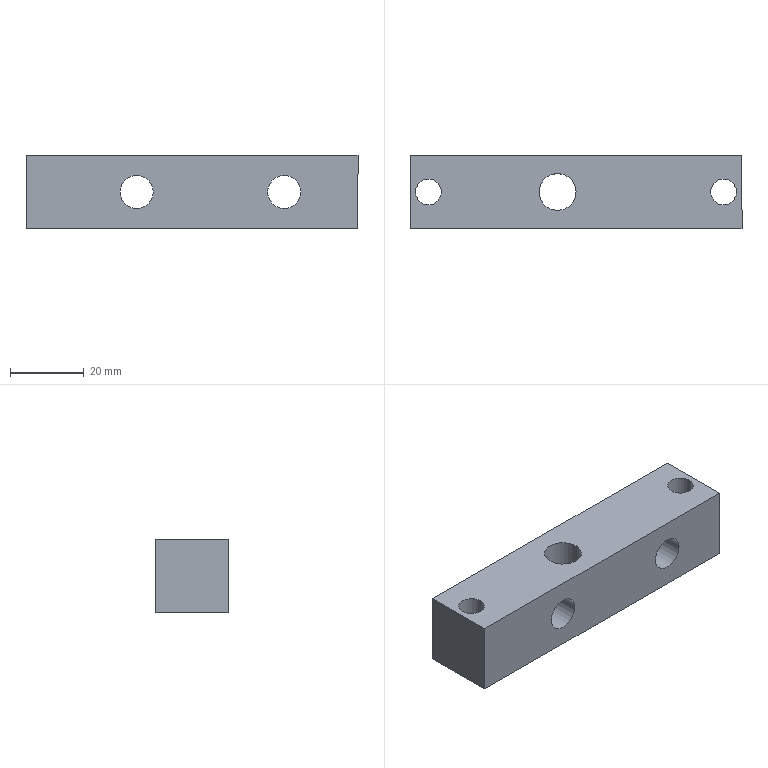Component | SolidWorks | CTM-T-12-AG-02-1 | 1 solid | 16 faces | box 90 x 20 x 20 mm | volume 30345 mm3 | cylinder 10 | plane 6 | commonest cylinder face diameters 7 x4 9 x4 10 x2 | material Q235A
build123d program:
from build123d import *

# Parameters (mm, degrees)
SKETCH1_W                = 20
SKETCH1_H                = 20
BOSS_EXTRUDE1_DEPTH      = 90
M8_CLEARANCE_HOLE1_D     = 9
M8_CLEARANCE_HOLE1_DEPTH = 20
M8_CLEARANCE_HOLE1_TIP   = 2.704
M10_TAPPED_HOLE1_D       = 10
M10_TAPPED_HOLE1_DEPTH   = 27.5
M10_TAPPED_HOLE1_TIP     = 3.004
M6_CLEARANCE_HOLE1_D     = 7
M6_CLEARANCE_HOLE1_DEPTH = 20
M6_CLEARANCE_HOLE1_TIP   = 2.103


with BuildPart() as part:
    # Sketch1 → Boss-Extrude1 (new body)
    with BuildSketch(Plane.XY):
        with Locations((10, 10)):
            Rectangle(SKETCH1_W, SKETCH1_H)
    extrude(amount=BOSS_EXTRUDE1_DEPTH)

    # M8 Clearance Hole1
    with Locations(Plane(origin=(0, 20, 0), x_dir=(-1, 0, 0), z_dir=(0, 1, 0))):
        with Locations((-10, 30), (-10, 70)):
            Hole(M8_CLEARANCE_HOLE1_D / 2, depth=M8_CLEARANCE_HOLE1_DEPTH)
            with Locations((0, 0, -(M8_CLEARANCE_HOLE1_DEPTH + M8_CLEARANCE_HOLE1_TIP / 2))):  # 118° drill point
                Cone(0, M8_CLEARANCE_HOLE1_D / 2, M8_CLEARANCE_HOLE1_TIP, mode=Mode.SUBTRACT)

    # M10 Tapped Hole1
    with Locations(Plane(origin=(20, 0, 0), x_dir=(0, 0, -1), z_dir=(1, 0, 0))):
        with Locations((-40, 10)):
            Hole(M10_TAPPED_HOLE1_D / 2, depth=M10_TAPPED_HOLE1_DEPTH)
            with Locations((0, 0, -(M10_TAPPED_HOLE1_DEPTH + M10_TAPPED_HOLE1_TIP / 2))):  # 118° drill point
                Cone(0, M10_TAPPED_HOLE1_D / 2, M10_TAPPED_HOLE1_TIP, mode=Mode.SUBTRACT)

    # M6 Clearance Hole1
    with Locations(Plane(origin=(20, 0, 0), x_dir=(0, 0, -1), z_dir=(1, 0, 0))):
        with Locations((-85, 10), (-5, 10)):
            Hole(M6_CLEARANCE_HOLE1_D / 2, depth=M6_CLEARANCE_HOLE1_DEPTH)
            with Locations((0, 0, -(M6_CLEARANCE_HOLE1_DEPTH + M6_CLEARANCE_HOLE1_TIP / 2))):  # 118° drill point
                Cone(0, M6_CLEARANCE_HOLE1_D / 2, M6_CLEARANCE_HOLE1_TIP, mode=Mode.SUBTRACT)


solid = part.part

# Placed as in the assembly
solid = solid.moved(Location((0.4, -20, 90), (0, 90, 0)))
STEP:
#1=COLOUR_RGB('',0.7922,0.8196,0.9333);
#2=FILL_AREA_STYLE_COLOUR('',#1);
#3=FILL_AREA_STYLE('',(#2));
#4=SURFACE_STYLE_FILL_AREA(#3);
#5=SURFACE_SIDE_STYLE('',(#4));
#6=SURFACE_STYLE_USAGE(.BOTH.,#5);
#7=PRESENTATION_STYLE_ASSIGNMENT((#6));
#8=CARTESIAN_POINT('',(3.5,-0.3937,2.756));
#9=VERTEX_POINT('',#8);
#10=CARTESIAN_POINT('',(3.224,-0.3937,2.756));
#11=VERTEX_POINT('',#10);
#12=CARTESIAN_POINT('',(3.362,-0.3937,2.756));
#13=DIRECTION('',(0.,-0.,1.));
#14=DIRECTION('',(-1.,0.,0.));
#15=AXIS2_PLACEMENT_3D('',#12,#13,#14);
#16=CIRCLE('',#15,0.1378);
#17=EDGE_CURVE('',#9,#11,#16,.T.);
#18=ORIENTED_EDGE('',*,*,#17,.F.);
#19=CARTESIAN_POINT('',(3.5,-0.3937,3.543));
#20=VERTEX_POINT('',#19);
#21=CARTESIAN_POINT('',(3.5,-0.3937,3.543));
#22=DIRECTION('',(0.,-0.,1.));
#23=VECTOR('',#22,39.37);
#24=LINE('',#21,#23);
#25=EDGE_CURVE('',#9,#20,#24,.T.);
#26=ORIENTED_EDGE('',*,*,#25,.T.);
#27=CARTESIAN_POINT('',(3.224,-0.3937,3.543));
#28=VERTEX_POINT('',#27);
#29=CARTESIAN_POINT('',(3.362,-0.3937,3.543));
#30=DIRECTION('',(0.,-0.,1.));
#31=DIRECTION('',(-1.,0.,0.));
#32=AXIS2_PLACEMENT_3D('',#29,#30,#31);
#33=CIRCLE('',#32,0.1378);
#34=EDGE_CURVE('',#20,#28,#33,.T.);
#35=ORIENTED_EDGE('',*,*,#34,.T.);
#36=CARTESIAN_POINT('',(3.224,-0.3937,3.543));
#37=DIRECTION('',(0.,-0.,1.));
#38=VECTOR('',#37,39.37);
#39=LINE('',#36,#38);
#40=EDGE_CURVE('',#11,#28,#39,.T.);
#41=ORIENTED_EDGE('',*,*,#40,.F.);
#42=EDGE_LOOP('',(#18,#26,#35,#41));
#43=FACE_OUTER_BOUND('',#42,.T.);
#44=CARTESIAN_POINT('',(3.362,-0.3937,3.543));
#45=DIRECTION('',(0.,-0.,1.));
#46=DIRECTION('',(-1.,0.,0.));
#47=AXIS2_PLACEMENT_3D('',#44,#45,#46);
#48=CYLINDRICAL_SURFACE('',#47,0.1378);
#49=ADVANCED_FACE('',(#43),#48,.F.);
#50=CARTESIAN_POINT('',(0.3504,-0.3937,2.756));
#51=VERTEX_POINT('',#50);
#52=CARTESIAN_POINT('',(0.0748,-0.3937,2.756));
#53=VERTEX_POINT('',#52);
#54=CARTESIAN_POINT('',(0.2126,-0.3937,2.756));
#55=DIRECTION('',(0.,-0.,1.));
#56=DIRECTION('',(-1.,0.,0.));
#57=AXIS2_PLACEMENT_3D('',#54,#55,#56);
#58=CIRCLE('',#57,0.1378);
#59=EDGE_CURVE('',#51,#53,#58,.T.);
#60=ORIENTED_EDGE('',*,*,#59,.F.);
#61=CARTESIAN_POINT('',(0.3504,-0.3937,3.543));
#62=VERTEX_POINT('',#61);
#63=CARTESIAN_POINT('',(0.3504,-0.3937,3.543));
#64=DIRECTION('',(0.,-0.,1.));
#65=VECTOR('',#64,39.37);
#66=LINE('',#63,#65);
#67=EDGE_CURVE('',#51,#62,#66,.T.);
#68=ORIENTED_EDGE('',*,*,#67,.T.);
#69=CARTESIAN_POINT('',(0.0748,-0.3937,3.543));
#70=VERTEX_POINT('',#69);
#71=CARTESIAN_POINT('',(0.2126,-0.3937,3.543));
#72=DIRECTION('',(0.,-0.,1.));
#73=DIRECTION('',(-1.,0.,0.));
#74=AXIS2_PLACEMENT_3D('',#71,#72,#73);
#75=CIRCLE('',#74,0.1378);
#76=EDGE_CURVE('',#62,#70,#75,.T.);
#77=ORIENTED_EDGE('',*,*,#76,.T.);
#78=CARTESIAN_POINT('',(0.0748,-0.3937,3.543));
#79=DIRECTION('',(0.,-0.,1.));
#80=VECTOR('',#79,39.37);
#81=LINE('',#78,#80);
#82=EDGE_CURVE('',#53,#70,#81,.T.);
#83=ORIENTED_EDGE('',*,*,#82,.F.);
#84=EDGE_LOOP('',(#60,#68,#77,#83));
#85=FACE_OUTER_BOUND('',#84,.T.);
#86=CARTESIAN_POINT('',(0.2126,-0.3937,3.543));
#87=DIRECTION('',(0.,-0.,1.));
#88=DIRECTION('',(-1.,0.,0.));
#89=AXIS2_PLACEMENT_3D('',#86,#87,#88);
#90=CYLINDRICAL_SURFACE('',#89,0.1378);
#91=ADVANCED_FACE('',(#85),#90,.F.);
#92=CARTESIAN_POINT('',(1.787,-0.3937,2.756));
#93=VERTEX_POINT('',#92);
#94=CARTESIAN_POINT('',(1.394,-0.3937,2.756));
#95=VERTEX_POINT('',#94);
#96=CARTESIAN_POINT('',(1.591,-0.3937,2.756));
#97=DIRECTION('',(0.,-0.,1.));
#98=DIRECTION('',(-1.,-0.,0.));
#99=AXIS2_PLACEMENT_3D('',#96,#97,#98);
#100=CIRCLE('',#99,0.1969);
#101=EDGE_CURVE('',#93,#95,#100,.T.);
#102=ORIENTED_EDGE('',*,*,#101,.F.);
#103=CARTESIAN_POINT('',(1.787,-0.3937,3.543));
#104=VERTEX_POINT('',#103);
#105=CARTESIAN_POINT('',(1.787,-0.3937,3.543));
#106=DIRECTION('',(0.,-0.,1.));
#107=VECTOR('',#106,39.37);
#108=LINE('',#105,#107);
#109=EDGE_CURVE('',#93,#104,#108,.T.);
#110=ORIENTED_EDGE('',*,*,#109,.T.);
#111=CARTESIAN_POINT('',(1.394,-0.3937,3.543));
#112=VERTEX_POINT('',#111);
#113=CARTESIAN_POINT('',(1.591,-0.3937,3.543));
#114=DIRECTION('',(0.,-0.,1.));
#115=DIRECTION('',(-1.,-0.,0.));
#116=AXIS2_PLACEMENT_3D('',#113,#114,#115);
#117=CIRCLE('',#116,0.1969);
#118=EDGE_CURVE('',#104,#112,#117,.T.);
#119=ORIENTED_EDGE('',*,*,#118,.T.);
#120=CARTESIAN_POINT('',(1.394,-0.3937,3.543));
#121=DIRECTION('',(0.,-0.,1.));
#122=VECTOR('',#121,39.37);
#123=LINE('',#120,#122);
#124=EDGE_CURVE('',#95,#112,#123,.T.);
#125=ORIENTED_EDGE('',*,*,#124,.F.);
#126=EDGE_LOOP('',(#102,#110,#119,#125));
#127=FACE_OUTER_BOUND('',#126,.T.);
#128=CARTESIAN_POINT('',(1.591,-0.3937,3.543));
#129=DIRECTION('',(0.,-0.,1.));
#130=DIRECTION('',(-1.,-0.,0.));
#131=AXIS2_PLACEMENT_3D('',#128,#129,#130);
#132=CYLINDRICAL_SURFACE('',#131,0.1969);
#133=ADVANCED_FACE('',(#127),#132,.F.);
#134=CARTESIAN_POINT('',(1.02,0.,3.15));
#135=VERTEX_POINT('',#134);
#136=CARTESIAN_POINT('',(1.374,0.,3.15));
#137=VERTEX_POINT('',#136);
#138=CARTESIAN_POINT('',(1.197,0.,3.15));
#139=DIRECTION('',(0.,-1.,-0.));
#140=DIRECTION('',(1.,0.,0.));
#141=AXIS2_PLACEMENT_3D('',#138,#139,#140);
#142=CIRCLE('',#141,0.1772);
#143=EDGE_CURVE('',#135,#137,#142,.T.);
#144=ORIENTED_EDGE('',*,*,#143,.F.);
#145=CARTESIAN_POINT('',(1.02,-0.7874,3.15));
#146=VERTEX_POINT('',#145);
#147=CARTESIAN_POINT('',(1.02,-0.7874,3.15));
#148=DIRECTION('',(0.,-1.,-0.));
#149=VECTOR('',#148,39.37);
#150=LINE('',#147,#149);
#151=EDGE_CURVE('',#135,#146,#150,.T.);
#152=ORIENTED_EDGE('',*,*,#151,.T.);
#153=CARTESIAN_POINT('',(1.374,-0.7874,3.15));
#154=VERTEX_POINT('',#153);
#155=CARTESIAN_POINT('',(1.197,-0.7874,3.15));
#156=DIRECTION('',(0.,-1.,-0.));
#157=DIRECTION('',(1.,0.,0.));
#158=AXIS2_PLACEMENT_3D('',#155,#156,#157);
#159=CIRCLE('',#158,0.1772);
#160=EDGE_CURVE('',#146,#154,#159,.T.);
#161=ORIENTED_EDGE('',*,*,#160,.T.);
#162=CARTESIAN_POINT('',(1.374,-0.7874,3.15));
#163=DIRECTION('',(0.,-1.,-0.));
#164=VECTOR('',#163,39.37);
#165=LINE('',#162,#164);
#166=EDGE_CURVE('',#137,#154,#165,.T.);
#167=ORIENTED_EDGE('',*,*,#166,.F.);
#168=EDGE_LOOP('',(#144,#152,#161,#167));
#169=FACE_OUTER_BOUND('',#168,.T.);
#170=CARTESIAN_POINT('',(1.197,-0.7874,3.15));
#171=DIRECTION('',(0.,-1.,-0.));
#172=DIRECTION('',(1.,0.,0.));
#173=AXIS2_PLACEMENT_3D('',#170,#171,#172);
#174=CYLINDRICAL_SURFACE('',#173,0.1772);
#175=ADVANCED_FACE('',(#169),#174,.F.);
#176=CARTESIAN_POINT('',(2.594,0.,3.15));
#177=VERTEX_POINT('',#176);
#178=CARTESIAN_POINT('',(2.949,0.,3.15));
#179=VERTEX_POINT('',#178);
#180=CARTESIAN_POINT('',(2.772,0.,3.15));
#181=DIRECTION('',(0.,-1.,-0.));
#182=DIRECTION('',(1.,0.,0.));
#183=AXIS2_PLACEMENT_3D('',#180,#181,#182);
#184=CIRCLE('',#183,0.1772);
#185=EDGE_CURVE('',#177,#179,#184,.T.);
#186=ORIENTED_EDGE('',*,*,#185,.F.);
#187=CARTESIAN_POINT('',(2.594,-0.7874,3.15));
#188=VERTEX_POINT('',#187);
#189=CARTESIAN_POINT('',(2.594,-0.7874,3.15));
#190=DIRECTION('',(0.,-1.,-0.));
#191=VECTOR('',#190,39.37);
#192=LINE('',#189,#191);
#193=EDGE_CURVE('',#177,#188,#192,.T.);
#194=ORIENTED_EDGE('',*,*,#193,.T.);
#195=CARTESIAN_POINT('',(2.949,-0.7874,3.15));
#196=VERTEX_POINT('',#195);
#197=CARTESIAN_POINT('',(2.772,-0.7874,3.15));
#198=DIRECTION('',(0.,-1.,-0.));
#199=DIRECTION('',(1.,0.,0.));
#200=AXIS2_PLACEMENT_3D('',#197,#198,#199);
#201=CIRCLE('',#200,0.1772);
#202=EDGE_CURVE('',#188,#196,#201,.T.);
#203=ORIENTED_EDGE('',*,*,#202,.T.);
#204=CARTESIAN_POINT('',(2.949,-0.7874,3.15));
#205=DIRECTION('',(0.,-1.,-0.));
#206=VECTOR('',#205,39.37);
#207=LINE('',#204,#206);
#208=EDGE_CURVE('',#179,#196,#207,.T.);
#209=ORIENTED_EDGE('',*,*,#208,.F.);
#210=EDGE_LOOP('',(#186,#194,#203,#209));
#211=FACE_OUTER_BOUND('',#210,.T.);
#212=CARTESIAN_POINT('',(2.772,-0.7874,3.15));
#213=DIRECTION('',(0.,-1.,-0.));
#214=DIRECTION('',(1.,0.,0.));
#215=AXIS2_PLACEMENT_3D('',#212,#213,#214);
#216=CYLINDRICAL_SURFACE('',#215,0.1772);
#217=ADVANCED_FACE('',(#211),#216,.F.);
#218=CARTESIAN_POINT('',(3.362,-0.3937,2.756));
#219=DIRECTION('',(0.,-0.,1.));
#220=DIRECTION('',(-1.,0.,0.));
#221=AXIS2_PLACEMENT_3D('',#218,#219,#220);
#222=CIRCLE('',#221,0.1378);
#223=EDGE_CURVE('',#11,#9,#222,.T.);
#224=ORIENTED_EDGE('',*,*,#223,.T.);
#225=ORIENTED_EDGE('',*,*,#17,.T.);
#226=EDGE_LOOP('',(#224,#225));
#227=FACE_BOUND('',#226,.T.);
#228=CARTESIAN_POINT('',(0.2126,-0.3937,2.756));
#229=DIRECTION('',(0.,-0.,1.));
#230=DIRECTION('',(-1.,0.,0.));
#231=AXIS2_PLACEMENT_3D('',#228,#229,#230);
#232=CIRCLE('',#231,0.1378);
#233=EDGE_CURVE('',#53,#51,#232,.T.);
#234=ORIENTED_EDGE('',*,*,#233,.T.);
#235=ORIENTED_EDGE('',*,*,#59,.T.);
#236=EDGE_LOOP('',(#234,#235));
#237=FACE_BOUND('',#236,.T.);
#238=CARTESIAN_POINT('',(1.591,-0.3937,2.756));
#239=DIRECTION('',(0.,-0.,1.));
#240=DIRECTION('',(-1.,-0.,0.));
#241=AXIS2_PLACEMENT_3D('',#238,#239,#240);
#242=CIRCLE('',#241,0.1969);
#243=EDGE_CURVE('',#95,#93,#242,.T.);
#244=ORIENTED_EDGE('',*,*,#243,.T.);
#245=ORIENTED_EDGE('',*,*,#101,.T.);
#246=EDGE_LOOP('',(#244,#245));
#247=FACE_BOUND('',#246,.T.);
#248=CARTESIAN_POINT('',(0.01575,-0.7874,2.756));
#249=VERTEX_POINT('',#248);
#250=CARTESIAN_POINT('',(0.01575,0.,2.756));
#251=VERTEX_POINT('',#250);
#252=CARTESIAN_POINT('',(0.01575,0.,2.756));
#253=DIRECTION('',(-0.,1.,0.));
#254=VECTOR('',#253,39.37);
#255=LINE('',#252,#254);
#256=EDGE_CURVE('',#249,#251,#255,.T.);
#257=ORIENTED_EDGE('',*,*,#256,.T.);
#258=CARTESIAN_POINT('',(3.559,0.,2.756));
#259=VERTEX_POINT('',#258);
#260=CARTESIAN_POINT('',(3.559,0.,2.756));
#261=DIRECTION('',(-1.,-0.,0.));
#262=VECTOR('',#261,39.37);
#263=LINE('',#260,#262);
#264=EDGE_CURVE('',#259,#251,#263,.T.);
#265=ORIENTED_EDGE('',*,*,#264,.F.);
#266=CARTESIAN_POINT('',(3.559,-0.7874,2.756));
#267=VERTEX_POINT('',#266);
#268=CARTESIAN_POINT('',(3.559,0.,2.756));
#269=DIRECTION('',(-0.,1.,0.));
#270=VECTOR('',#269,39.37);
#271=LINE('',#268,#270);
#272=EDGE_CURVE('',#267,#259,#271,.T.);
#273=ORIENTED_EDGE('',*,*,#272,.F.);
#274=CARTESIAN_POINT('',(3.559,-0.7874,2.756));
#275=DIRECTION('',(-1.,-0.,0.));
#276=VECTOR('',#275,39.37);
#277=LINE('',#274,#276);
#278=EDGE_CURVE('',#267,#249,#277,.T.);
#279=ORIENTED_EDGE('',*,*,#278,.T.);
#280=EDGE_LOOP('',(#257,#265,#273,#279));
#281=FACE_OUTER_BOUND('',#280,.T.);
#282=CARTESIAN_POINT('',(3.559,0.,2.756));
#283=DIRECTION('',(0.,-0.,1.));
#284=DIRECTION('',(-1.,-0.,0.));
#285=AXIS2_PLACEMENT_3D('',#282,#283,#284);
#286=PLANE('',#285);
#287=ADVANCED_FACE('',(#227,#237,#247,#281),#286,.F.);
#288=CARTESIAN_POINT('',(1.197,0.,3.15));
#289=DIRECTION('',(0.,-1.,-0.));
#290=DIRECTION('',(1.,0.,0.));
#291=AXIS2_PLACEMENT_3D('',#288,#289,#290);
#292=CIRCLE('',#291,0.1772);
#293=EDGE_CURVE('',#137,#135,#292,.T.);
#294=ORIENTED_EDGE('',*,*,#293,.T.);
#295=ORIENTED_EDGE('',*,*,#143,.T.);
#296=EDGE_LOOP('',(#294,#295));
#297=FACE_BOUND('',#296,.T.);
#298=CARTESIAN_POINT('',(2.772,0.,3.15));
#299=DIRECTION('',(0.,-1.,-0.));
#300=DIRECTION('',(1.,0.,0.));
#301=AXIS2_PLACEMENT_3D('',#298,#299,#300);
#302=CIRCLE('',#301,0.1772);
#303=EDGE_CURVE('',#179,#177,#302,.T.);
#304=ORIENTED_EDGE('',*,*,#303,.T.);
#305=ORIENTED_EDGE('',*,*,#185,.T.);
#306=EDGE_LOOP('',(#304,#305));
#307=FACE_BOUND('',#306,.T.);
#308=CARTESIAN_POINT('',(0.01575,0.,3.543));
#309=VERTEX_POINT('',#308);
#310=CARTESIAN_POINT('',(0.01575,0.,2.756));
#311=DIRECTION('',(0.,-0.,1.));
#312=VECTOR('',#311,39.37);
#313=LINE('',#310,#312);
#314=EDGE_CURVE('',#251,#309,#313,.T.);
#315=ORIENTED_EDGE('',*,*,#314,.T.);
#316=CARTESIAN_POINT('',(3.559,0.,3.543));
#317=VERTEX_POINT('',#316);
#318=CARTESIAN_POINT('',(3.559,0.,3.543));
#319=DIRECTION('',(-1.,-0.,0.));
#320=VECTOR('',#319,39.37);
#321=LINE('',#318,#320);
#322=EDGE_CURVE('',#317,#309,#321,.T.);
#323=ORIENTED_EDGE('',*,*,#322,.F.);
#324=CARTESIAN_POINT('',(3.559,0.,2.756));
#325=DIRECTION('',(0.,-0.,1.));
#326=VECTOR('',#325,39.37);
#327=LINE('',#324,#326);
#328=EDGE_CURVE('',#259,#317,#327,.T.);
#329=ORIENTED_EDGE('',*,*,#328,.F.);
#330=ORIENTED_EDGE('',*,*,#264,.T.);
#331=EDGE_LOOP('',(#315,#323,#329,#330));
#332=FACE_OUTER_BOUND('',#331,.T.);
#333=CARTESIAN_POINT('',(3.559,0.,2.756));
#334=DIRECTION('',(0.,-1.,-0.));
#335=DIRECTION('',(1.,0.,-0.));
#336=AXIS2_PLACEMENT_3D('',#333,#334,#335);
#337=PLANE('',#336);
#338=ADVANCED_FACE('',(#297,#307,#332),#337,.F.);
#339=CARTESIAN_POINT('',(3.362,-0.3937,3.543));
#340=DIRECTION('',(0.,-0.,1.));
#341=DIRECTION('',(-1.,0.,0.));
#342=AXIS2_PLACEMENT_3D('',#339,#340,#341);
#343=CIRCLE('',#342,0.1378);
#344=EDGE_CURVE('',#28,#20,#343,.T.);
#345=ORIENTED_EDGE('',*,*,#344,.F.);
#346=ORIENTED_EDGE('',*,*,#34,.F.);
#347=EDGE_LOOP('',(#345,#346));
#348=FACE_BOUND('',#347,.T.);
#349=CARTESIAN_POINT('',(0.2126,-0.3937,3.543));
#350=DIRECTION('',(0.,-0.,1.));
#351=DIRECTION('',(-1.,0.,0.));
#352=AXIS2_PLACEMENT_3D('',#349,#350,#351);
#353=CIRCLE('',#352,0.1378);
#354=EDGE_CURVE('',#70,#62,#353,.T.);
#355=ORIENTED_EDGE('',*,*,#354,.F.);
#356=ORIENTED_EDGE('',*,*,#76,.F.);
#357=EDGE_LOOP('',(#355,#356));
#358=FACE_BOUND('',#357,.T.);
#359=CARTESIAN_POINT('',(1.591,-0.3937,3.543));
#360=DIRECTION('',(0.,-0.,1.));
#361=DIRECTION('',(-1.,-0.,0.));
#362=AXIS2_PLACEMENT_3D('',#359,#360,#361);
#363=CIRCLE('',#362,0.1969);
#364=EDGE_CURVE('',#112,#104,#363,.T.);
#365=ORIENTED_EDGE('',*,*,#364,.F.);
#366=ORIENTED_EDGE('',*,*,#118,.F.);
#367=EDGE_LOOP('',(#365,#366));
#368=FACE_BOUND('',#367,.T.);
#369=CARTESIAN_POINT('',(0.01575,-0.7874,3.543));
#370=VERTEX_POINT('',#369);
#371=CARTESIAN_POINT('',(0.01575,0.,3.543));
#372=DIRECTION('',(0.,-1.,-0.));
#373=VECTOR('',#372,39.37);
#374=LINE('',#371,#373);
#375=EDGE_CURVE('',#309,#370,#374,.T.);
#376=ORIENTED_EDGE('',*,*,#375,.T.);
#377=CARTESIAN_POINT('',(3.559,-0.7874,3.543));
#378=VERTEX_POINT('',#377);
#379=CARTESIAN_POINT('',(3.559,-0.7874,3.543));
#380=DIRECTION('',(-1.,-0.,0.));
#381=VECTOR('',#380,39.37);
#382=LINE('',#379,#381);
#383=EDGE_CURVE('',#378,#370,#382,.T.);
#384=ORIENTED_EDGE('',*,*,#383,.F.);
#385=CARTESIAN_POINT('',(3.559,0.,3.543));
#386=DIRECTION('',(0.,-1.,-0.));
#387=VECTOR('',#386,39.37);
#388=LINE('',#385,#387);
#389=EDGE_CURVE('',#317,#378,#388,.T.);
#390=ORIENTED_EDGE('',*,*,#389,.F.);
#391=ORIENTED_EDGE('',*,*,#322,.T.);
#392=EDGE_LOOP('',(#376,#384,#390,#391));
#393=FACE_OUTER_BOUND('',#392,.T.);
#394=CARTESIAN_POINT('',(3.559,0.,3.543));
#395=DIRECTION('',(-0.,0.,-1.));
#396=DIRECTION('',(-0.,1.,0.));
#397=AXIS2_PLACEMENT_3D('',#394,#395,#396);
#398=PLANE('',#397);
#399=ADVANCED_FACE('',(#348,#358,#368,#393),#398,.F.);
#400=CARTESIAN_POINT('',(1.197,-0.7874,3.15));
#401=DIRECTION('',(0.,-1.,-0.));
#402=DIRECTION('',(1.,0.,0.));
#403=AXIS2_PLACEMENT_3D('',#400,#401,#402);
#404=CIRCLE('',#403,0.1772);
#405=EDGE_CURVE('',#154,#146,#404,.T.);
#406=ORIENTED_EDGE('',*,*,#405,.F.);
#407=ORIENTED_EDGE('',*,*,#160,.F.);
#408=EDGE_LOOP('',(#406,#407));
#409=FACE_BOUND('',#408,.T.);
#410=CARTESIAN_POINT('',(2.772,-0.7874,3.15));
#411=DIRECTION('',(0.,-1.,-0.));
#412=DIRECTION('',(1.,0.,0.));
#413=AXIS2_PLACEMENT_3D('',#410,#411,#412);
#414=CIRCLE('',#413,0.1772);
#415=EDGE_CURVE('',#196,#188,#414,.T.);
#416=ORIENTED_EDGE('',*,*,#415,.F.);
#417=ORIENTED_EDGE('',*,*,#202,.F.);
#418=EDGE_LOOP('',(#416,#417));
#419=FACE_BOUND('',#418,.T.);
#420=CARTESIAN_POINT('',(0.01575,-0.7874,2.756));
#421=DIRECTION('',(-0.,0.,-1.));
#422=VECTOR('',#421,39.37);
#423=LINE('',#420,#422);
#424=EDGE_CURVE('',#370,#249,#423,.T.);
#425=ORIENTED_EDGE('',*,*,#424,.T.);
#426=ORIENTED_EDGE('',*,*,#278,.F.);
#427=CARTESIAN_POINT('',(3.559,-0.7874,2.756));
#428=DIRECTION('',(-0.,0.,-1.));
#429=VECTOR('',#428,39.37);
#430=LINE('',#427,#429);
#431=EDGE_CURVE('',#378,#267,#430,.T.);
#432=ORIENTED_EDGE('',*,*,#431,.F.);
#433=ORIENTED_EDGE('',*,*,#383,.T.);
#434=EDGE_LOOP('',(#425,#426,#432,#433));
#435=FACE_OUTER_BOUND('',#434,.T.);
#436=CARTESIAN_POINT('',(3.559,-0.7874,2.756));
#437=DIRECTION('',(-0.,1.,0.));
#438=DIRECTION('',(-1.,-0.,0.));
#439=AXIS2_PLACEMENT_3D('',#436,#437,#438);
#440=PLANE('',#439);
#441=ADVANCED_FACE('',(#409,#419,#435),#440,.F.);
#442=ORIENTED_EDGE('',*,*,#272,.T.);
#443=ORIENTED_EDGE('',*,*,#328,.T.);
#444=ORIENTED_EDGE('',*,*,#389,.T.);
#445=ORIENTED_EDGE('',*,*,#431,.T.);
#446=EDGE_LOOP('',(#442,#443,#444,#445));
#447=FACE_OUTER_BOUND('',#446,.T.);
#448=CARTESIAN_POINT('',(3.559,-0.7874,2.756));
#449=DIRECTION('',(-1.,-0.,0.));
#450=DIRECTION('',(-0.,0.,-1.));
#451=AXIS2_PLACEMENT_3D('',#448,#449,#450);
#452=PLANE('',#451);
#453=ADVANCED_FACE('',(#447),#452,.F.);
#454=ORIENTED_EDGE('',*,*,#256,.F.);
#455=ORIENTED_EDGE('',*,*,#424,.F.);
#456=ORIENTED_EDGE('',*,*,#375,.F.);
#457=ORIENTED_EDGE('',*,*,#314,.F.);
#458=EDGE_LOOP('',(#454,#455,#456,#457));
#459=FACE_OUTER_BOUND('',#458,.T.);
#460=CARTESIAN_POINT('',(0.01575,-0.7874,2.756));
#461=DIRECTION('',(-1.,-0.,0.));
#462=DIRECTION('',(-0.,0.,-1.));
#463=AXIS2_PLACEMENT_3D('',#460,#461,#462);
#464=PLANE('',#463);
#465=ADVANCED_FACE('',(#459),#464,.T.);
#466=ORIENTED_EDGE('',*,*,#193,.F.);
#467=ORIENTED_EDGE('',*,*,#303,.F.);
#468=ORIENTED_EDGE('',*,*,#208,.T.);
#469=ORIENTED_EDGE('',*,*,#415,.T.);
#470=EDGE_LOOP('',(#466,#467,#468,#469));
#471=FACE_OUTER_BOUND('',#470,.T.);
#472=CARTESIAN_POINT('',(2.772,-0.7874,3.15));
#473=DIRECTION('',(0.,-1.,-0.));
#474=DIRECTION('',(1.,0.,0.));
#475=AXIS2_PLACEMENT_3D('',#472,#473,#474);
#476=CYLINDRICAL_SURFACE('',#475,0.1772);
#477=ADVANCED_FACE('',(#471),#476,.F.);
#478=ORIENTED_EDGE('',*,*,#151,.F.);
#479=ORIENTED_EDGE('',*,*,#293,.F.);
#480=ORIENTED_EDGE('',*,*,#166,.T.);
#481=ORIENTED_EDGE('',*,*,#405,.T.);
#482=EDGE_LOOP('',(#478,#479,#480,#481));
#483=FACE_OUTER_BOUND('',#482,.T.);
#484=CARTESIAN_POINT('',(1.197,-0.7874,3.15));
#485=DIRECTION('',(0.,-1.,-0.));
#486=DIRECTION('',(1.,0.,0.));
#487=AXIS2_PLACEMENT_3D('',#484,#485,#486);
#488=CYLINDRICAL_SURFACE('',#487,0.1772);
#489=ADVANCED_FACE('',(#483),#488,.F.);
#490=ORIENTED_EDGE('',*,*,#109,.F.);
#491=ORIENTED_EDGE('',*,*,#243,.F.);
#492=ORIENTED_EDGE('',*,*,#124,.T.);
#493=ORIENTED_EDGE('',*,*,#364,.T.);
#494=EDGE_LOOP('',(#490,#491,#492,#493));
#495=FACE_OUTER_BOUND('',#494,.T.);
#496=CARTESIAN_POINT('',(1.591,-0.3937,3.543));
#497=DIRECTION('',(0.,-0.,1.));
#498=DIRECTION('',(-1.,-0.,0.));
#499=AXIS2_PLACEMENT_3D('',#496,#497,#498);
#500=CYLINDRICAL_SURFACE('',#499,0.1969);
#501=ADVANCED_FACE('',(#495),#500,.F.);
#502=ORIENTED_EDGE('',*,*,#67,.F.);
#503=ORIENTED_EDGE('',*,*,#233,.F.);
#504=ORIENTED_EDGE('',*,*,#82,.T.);
#505=ORIENTED_EDGE('',*,*,#354,.T.);
#506=EDGE_LOOP('',(#502,#503,#504,#505));
#507=FACE_OUTER_BOUND('',#506,.T.);
#508=CARTESIAN_POINT('',(0.2126,-0.3937,3.543));
#509=DIRECTION('',(0.,-0.,1.));
#510=DIRECTION('',(-1.,0.,0.));
#511=AXIS2_PLACEMENT_3D('',#508,#509,#510);
#512=CYLINDRICAL_SURFACE('',#511,0.1378);
#513=ADVANCED_FACE('',(#507),#512,.F.);
#514=ORIENTED_EDGE('',*,*,#25,.F.);
#515=ORIENTED_EDGE('',*,*,#223,.F.);
#516=ORIENTED_EDGE('',*,*,#40,.T.);
#517=ORIENTED_EDGE('',*,*,#344,.T.);
#518=EDGE_LOOP('',(#514,#515,#516,#517));
#519=FACE_OUTER_BOUND('',#518,.T.);
#520=CARTESIAN_POINT('',(3.362,-0.3937,3.543));
#521=DIRECTION('',(0.,-0.,1.));
#522=DIRECTION('',(-1.,0.,0.));
#523=AXIS2_PLACEMENT_3D('',#520,#521,#522);
#524=CYLINDRICAL_SURFACE('',#523,0.1378);
#525=ADVANCED_FACE('',(#519),#524,.F.);
#526=CLOSED_SHELL('',(#49,#91,#133,#175,#217,#287,#338,#399,#441,#453,#465,#477,#489,#501,#513,#525));
#527=MANIFOLD_SOLID_BREP('',#526);
#528=STYLED_ITEM('',(#7),#527);
#529=PRESENTATION_LAYER_ASSIGNMENT('','',(#528));
#530=CARTESIAN_POINT('',(0.,0.,0.));
#531=DIRECTION('',(0.,0.,1.));
#532=DIRECTION('',(1.,0.,0.));
#533=AXIS2_PLACEMENT_3D('',#530,#531,#532);
#534=(LENGTH_UNIT()NAMED_UNIT(*)SI_UNIT($,.METRE.));
#535=LENGTH_MEASURE_WITH_UNIT(LENGTH_MEASURE(0.0254),#534);
#536=DIMENSIONAL_EXPONENTS(1.,0.,0.,0.,0.,0.,0.);
#537=(CONVERSION_BASED_UNIT('',#535)LENGTH_UNIT()NAMED_UNIT(#536));
#538=UNCERTAINTY_MEASURE_WITH_UNIT(LENGTH_MEASURE(0.00001),#537,'','');
#539=(NAMED_UNIT(*)PLANE_ANGLE_UNIT()SI_UNIT($,.RADIAN.));
#540=(NAMED_UNIT(*)SI_UNIT($,.STERADIAN.)SOLID_ANGLE_UNIT());
#541=(GEOMETRIC_REPRESENTATION_CONTEXT(3)GLOBAL_UNCERTAINTY_ASSIGNED_CONTEXT((#538))GLOBAL_UNIT_ASSIGNED_CONTEXT((#537,#539,#540))REPRESENTATION_CONTEXT('',''));
#542=ADVANCED_BREP_SHAPE_REPRESENTATION('',(#527,#533),#541);
#543=(LENGTH_UNIT()NAMED_UNIT(*)SI_UNIT($,.METRE.));
#544=LENGTH_MEASURE_WITH_UNIT(LENGTH_MEASURE(0.0254),#543);
#545=DIMENSIONAL_EXPONENTS(1.,0.,0.,0.,0.,0.,0.);
#546=(CONVERSION_BASED_UNIT('',#544)LENGTH_UNIT()NAMED_UNIT(#545));
#547=UNCERTAINTY_MEASURE_WITH_UNIT(LENGTH_MEASURE(0.00001),#546,'','');
#548=(NAMED_UNIT(*)PLANE_ANGLE_UNIT()SI_UNIT($,.RADIAN.));
#549=(NAMED_UNIT(*)SI_UNIT($,.STERADIAN.)SOLID_ANGLE_UNIT());
#550=(GEOMETRIC_REPRESENTATION_CONTEXT(3)GLOBAL_UNCERTAINTY_ASSIGNED_CONTEXT((#547))GLOBAL_UNIT_ASSIGNED_CONTEXT((#546,#548,#549))REPRESENTATION_CONTEXT('',''));
#551=MECHANICAL_DESIGN_GEOMETRIC_PRESENTATION_REPRESENTATION('',(#528),#550);